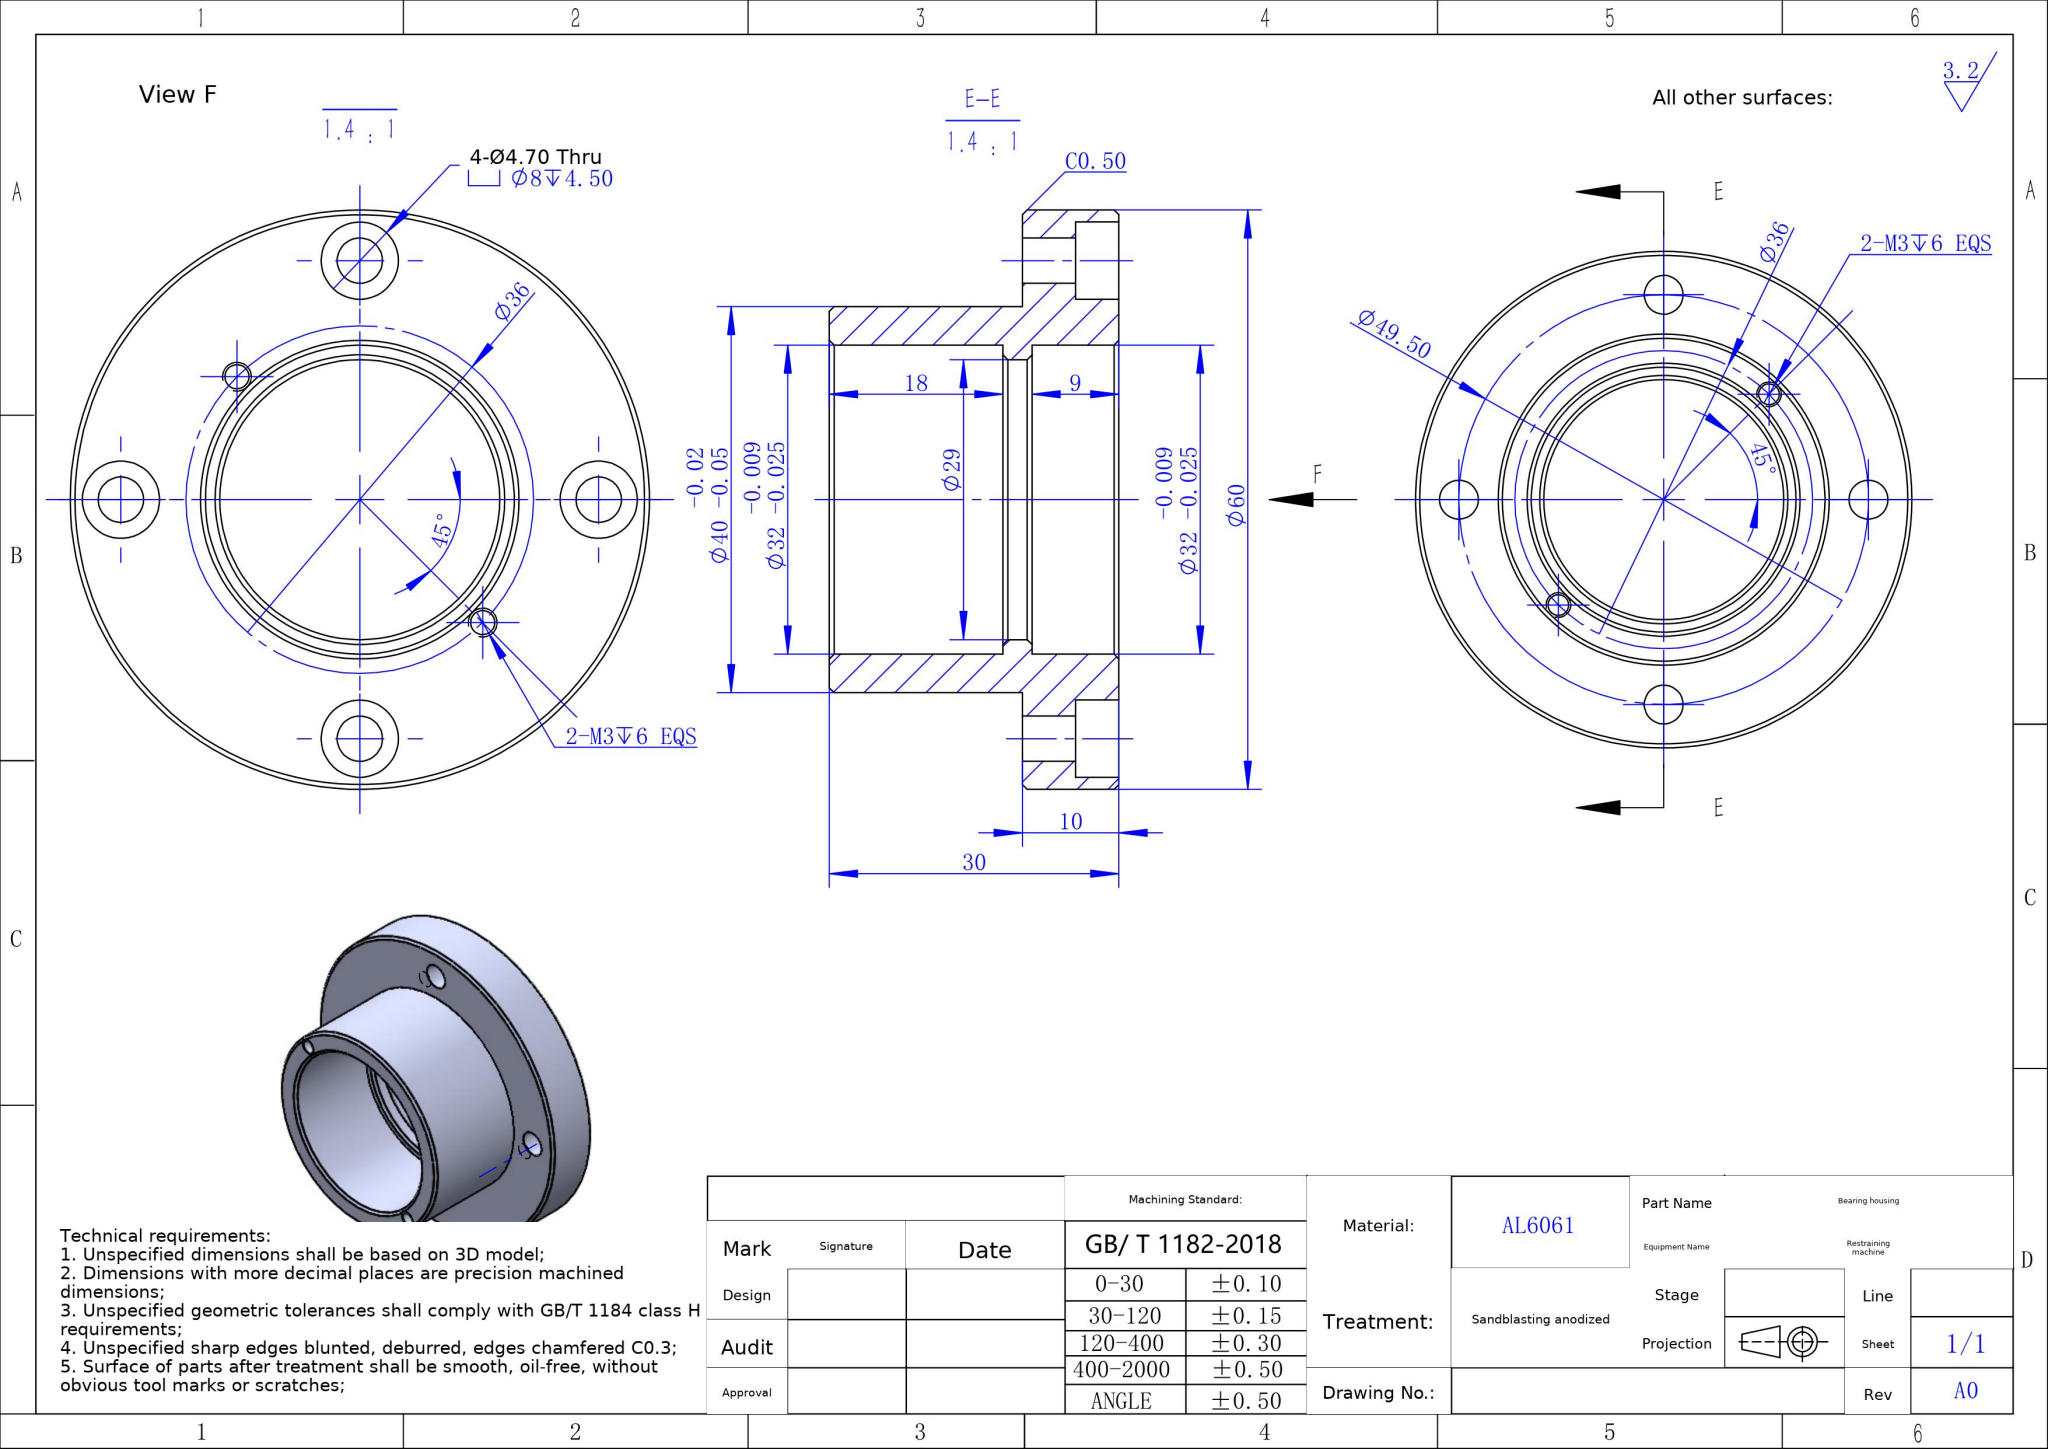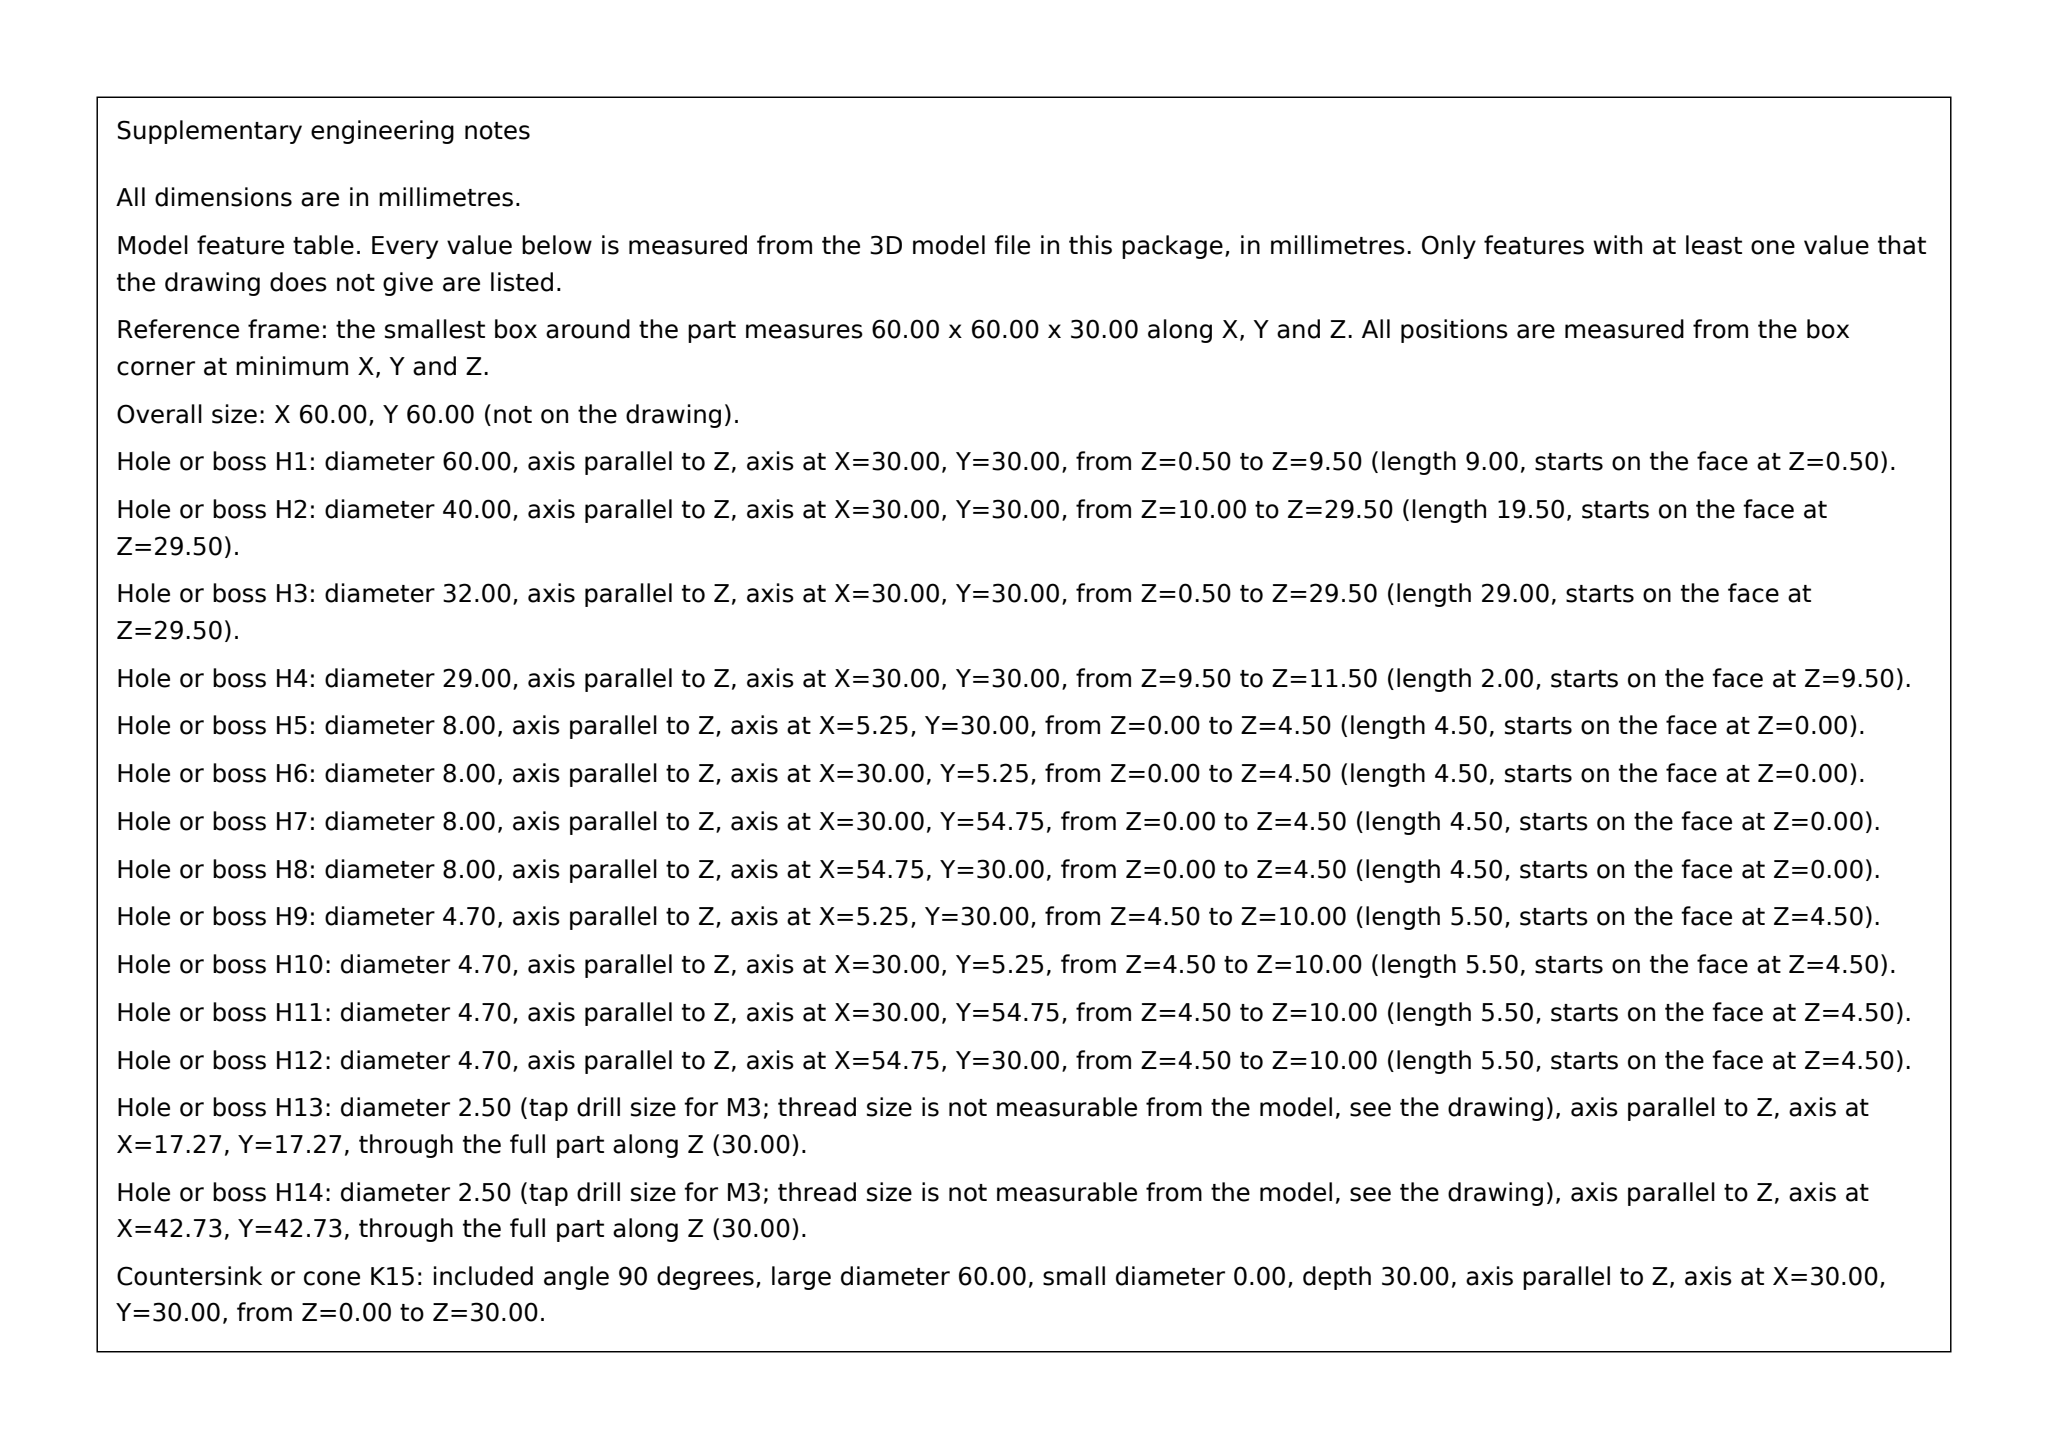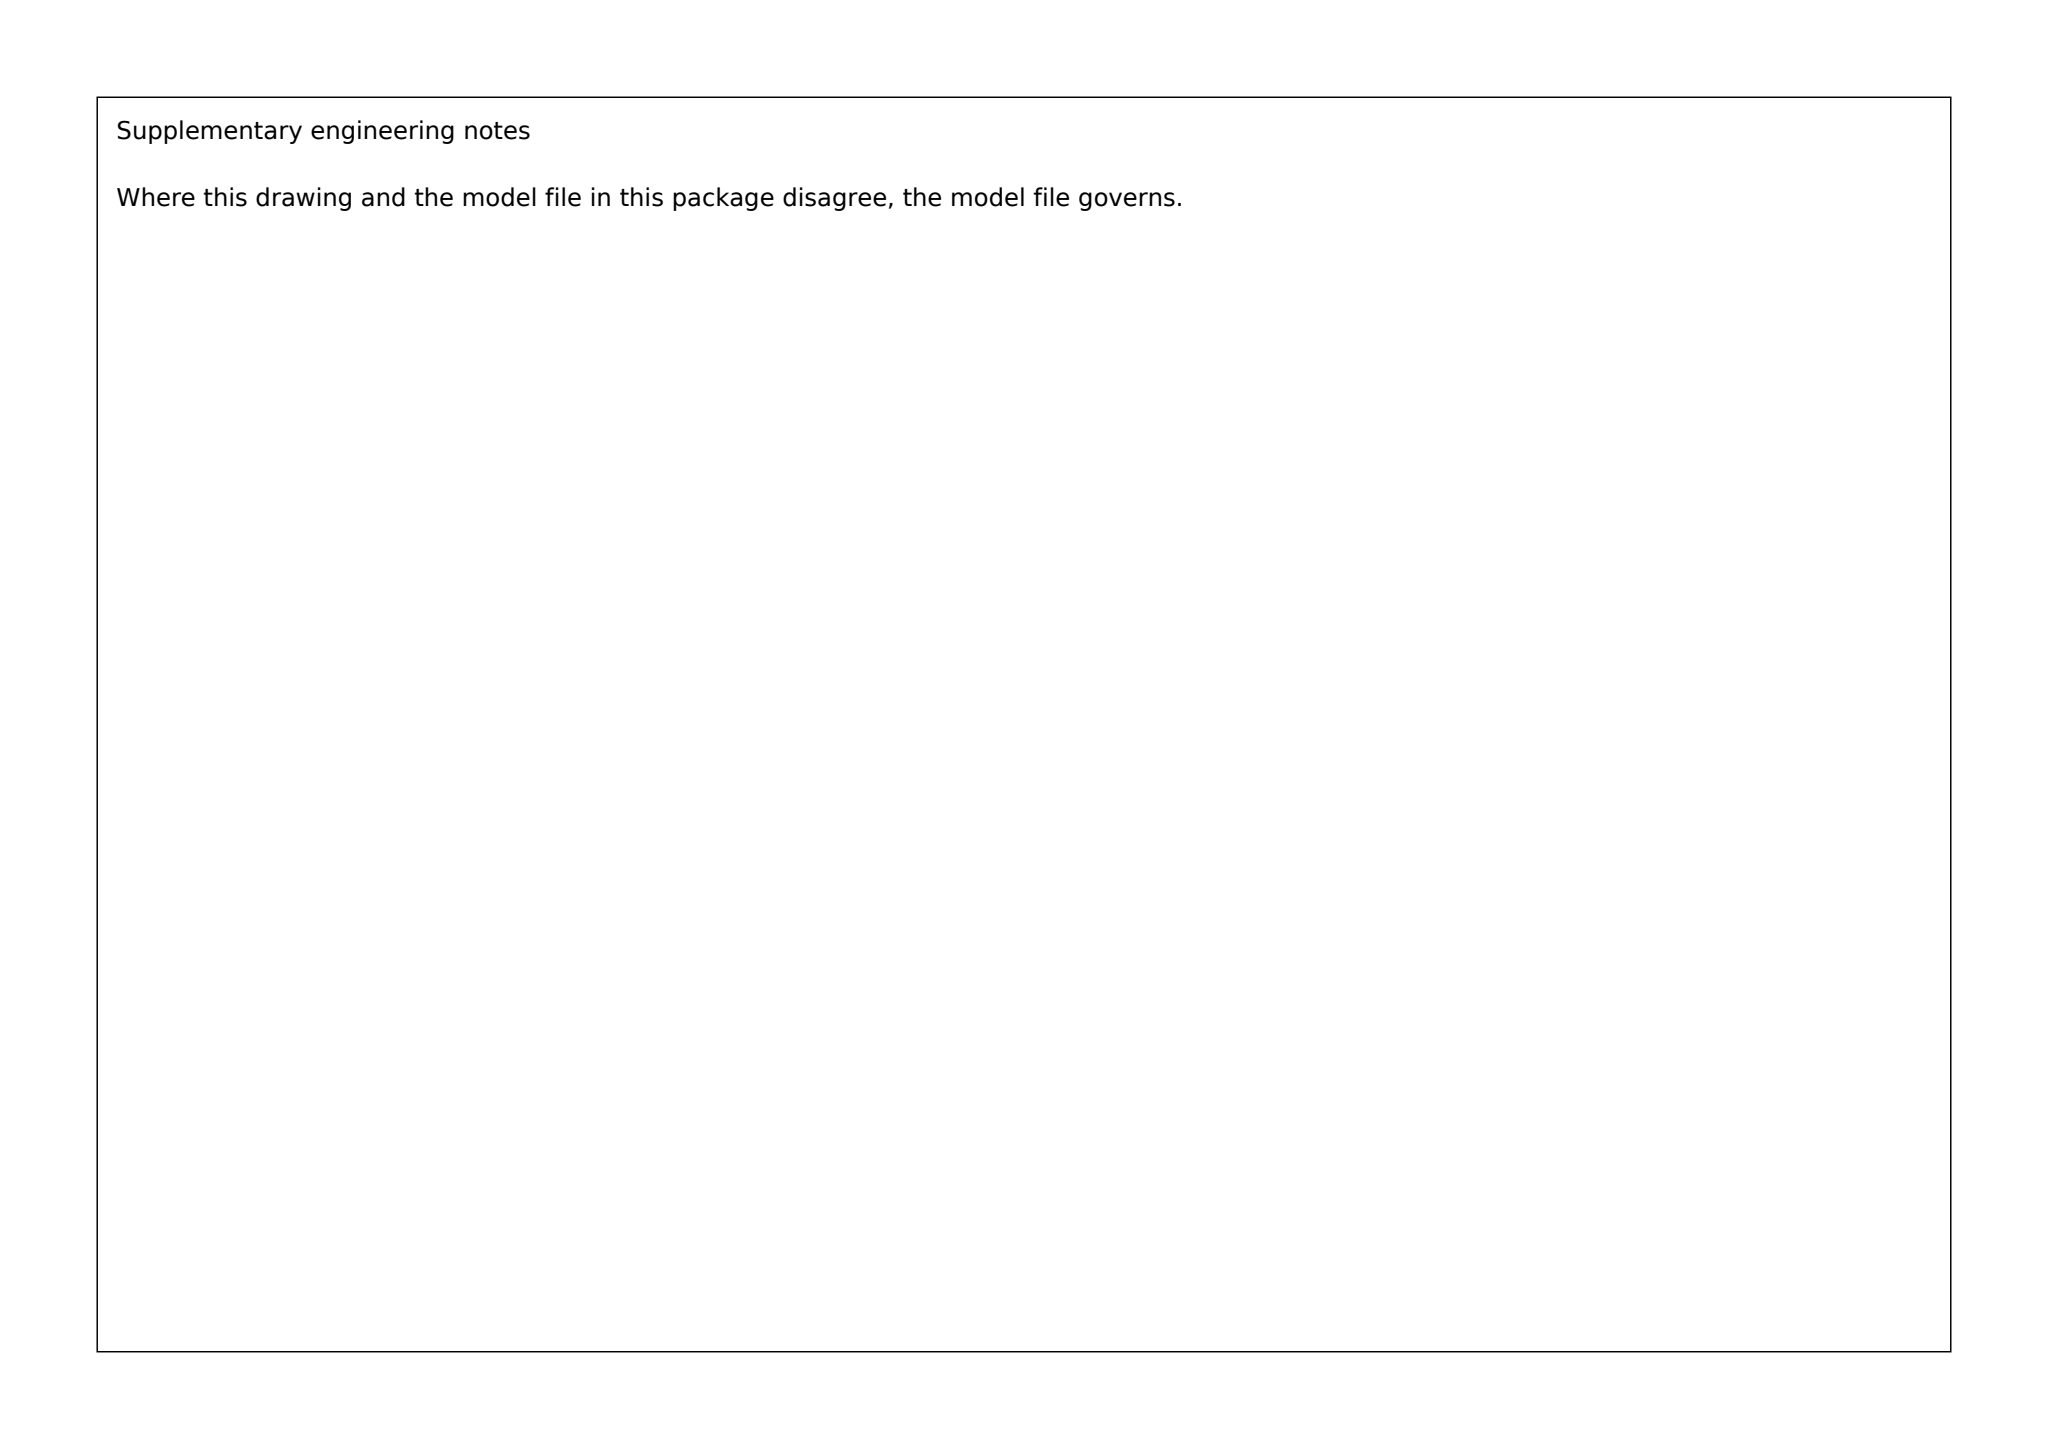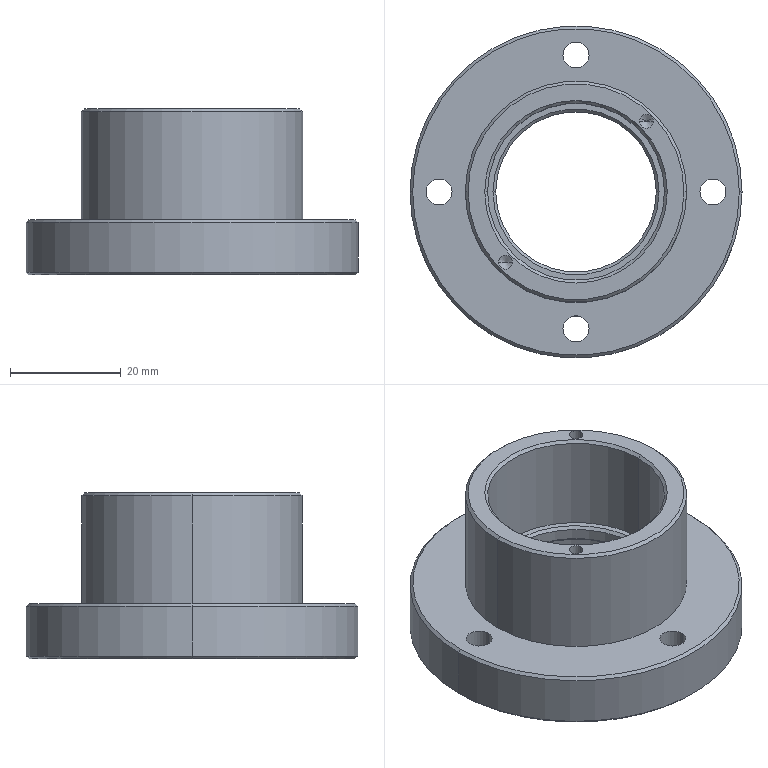Part | SolidWorks | mm | material AL6061 | 1 solid | 65 faces | box 60 x 60 x 30 mm | volume 28142 mm3 | cylinder 34 | cone 22 | plane 9 | commonest cylinder face diameters 2.5 x8 8 x8 4.7 x8 32 x4 40 x2 60 x2 29 x2
build123d program:
from build123d import *

# Parameters (mm, degrees)
SKETCH1_R                  = 30
BOSS_EXTRUDE1_DEPTH        = 10
SKETCH2_R                  = 20
BOSS_EXTRUDE2_DEPTH        = 20
SKETCH3_R                  = 14.5
CUT_EXTRUDE1_DEPTH         = 35
SKETCH4_R                  = 16
CUT_EXTRUDE2_DEPTH         = 9
CUT_EXTRUDE3_START         = -18
SKETCH5_R                  = 16
CUT_EXTRUDE3_DEPTH         = 18
CHAMFER1_SIZE              = 0.5
SKETCH6_R                  = 2.35
CUT_EXTRUDE4_DEPTH         = 18
SKETCH7_R                  = 4
CUT_EXTRUDE5_DEPTH         = 4.5
M3_TAPPED_HOLE2_AT_2_COUNT = 2
M3_TAPPED_HOLE2_AT_2_PITCH = 36


with BuildPart() as part:
    # Sketch1 → Boss-Extrude1 (new body)
    with BuildSketch(Plane.XY):
        Circle(SKETCH1_R)
    extrude(amount=BOSS_EXTRUDE1_DEPTH)

    # Sketch2 → Boss-Extrude2 (add)
    with BuildSketch(Plane.XY.offset(10)):
        Circle(SKETCH2_R)
    extrude(amount=BOSS_EXTRUDE2_DEPTH)

    # Sketch3 → Cut-Extrude1 (cut, symmetric)
    with BuildSketch(Plane(origin=(0, 0, 0), x_dir=(-1, 0, 0), z_dir=(0, 0, -1))):
        with Locations(Location((0, 0, 0), (0, 0, 180))):
            Circle(SKETCH3_R)
    extrude(amount=CUT_EXTRUDE1_DEPTH, both=True, mode=Mode.SUBTRACT)

    # Sketch4 → Cut-Extrude2 (cut)
    with BuildSketch(Plane(origin=(0, 0, 0), x_dir=(-1, 0, 0), z_dir=(0, 0, -1))):
        Circle(SKETCH4_R)
    extrude(amount=-CUT_EXTRUDE2_DEPTH, mode=Mode.SUBTRACT)

    # Sketch5 → Cut-Extrude3 (cut)
    with BuildSketch(Plane.XY.offset(30).offset(CUT_EXTRUDE3_START)):
        with Locations(Location((0, 0, 0), (0, 0, 180))):
            Circle(SKETCH5_R)
    extrude(amount=CUT_EXTRUDE3_DEPTH, mode=Mode.SUBTRACT)

    # Chamfer1
    chamfer1_edges = [part.edges().sort_by_distance(p)[0] for p in [
        (16, 0, 0),
        (-14.5, 0, 9),
        (-30, 0, 0),
        (16, 0, 30),
        (-14.5, 0, 12),
        (-30, 0, 10),
        (-20, 0, 30),
    ]]
    chamfer(chamfer1_edges, length=CHAMFER1_SIZE)

    # Sketch6 → Cut-Extrude4 (cut)
    with BuildSketch(Plane(origin=(0, 0, 0), x_dir=(-1, 0, 0), z_dir=(0, 0, -1))):
        with Locations((0, 24.75)):
            Circle(SKETCH6_R)
        with Locations((24.75, 0)):
            Circle(SKETCH6_R)
        with Locations((0, -24.75)):
            Circle(SKETCH6_R)
        with Locations((-24.75, 0)):
            Circle(SKETCH6_R)
    extrude(amount=-CUT_EXTRUDE4_DEPTH, mode=Mode.SUBTRACT)

    # Sketch7 → Cut-Extrude5 (cut)
    with BuildSketch(Plane(origin=(0, 0, 0), x_dir=(-1, 0, 0), z_dir=(0, 0, -1))):
        with Locations((0, 24.75)):
            Circle(SKETCH7_R)
        with Locations((0, -24.75)):
            Circle(SKETCH7_R)
        with Locations((-24.75, 0)):
            Circle(SKETCH7_R)
        with Locations((24.75, 0)):
            Circle(SKETCH7_R)
    extrude(amount=-CUT_EXTRUDE5_DEPTH, mode=Mode.SUBTRACT)

    # Sketch9 → M3 Tapped Hole2 (revolve, cut)
    with BuildSketch(Plane(origin=(-12.728, -12.728, 0), x_dir=(0, 1, 0), z_dir=(1, 0, 0))):
        Polygon((0, 0), (0, 9.251), (1.25, 8.5), (1.25, 0), align=None)
    m3_tapped_hole2 = revolve(axis=Axis((-12.728, -12.728, -6.35), (0, 0, 1)), mode=Mode.SUBTRACT)

    # M3 Tapped Hole2 at 2: M3 Tapped Hole2 ×2
    with Locations(*[Vector(0.7071, 0.7071, 0) * (i * M3_TAPPED_HOLE2_AT_2_PITCH) for i in range(1, M3_TAPPED_HOLE2_AT_2_COUNT)]):
        add(m3_tapped_hole2, mode=Mode.SUBTRACT)

    # Mirror1: M3 Tapped Hole2 across plane
    add(m3_tapped_hole2.mirror(Plane(origin=(0, 0, 15), x_dir=(1, 0, 0), z_dir=(0, 0, -1))), mode=Mode.SUBTRACT)

    # Mirror1 copy 1 sketch → Mirror1 copy 1 (revolve, cut)
    with BuildSketch(Plane(origin=(12.728, 12.728, 30), x_dir=(0, 1, 0), z_dir=(1, 0, 0))):
        Polygon((0, 0), (0, -9.251), (1.25, -8.5), (1.25, 0), align=None)
    revolve(axis=Axis((12.728, 12.728, 36.35), (0, 0, 1)), mode=Mode.SUBTRACT)


solid = part.part